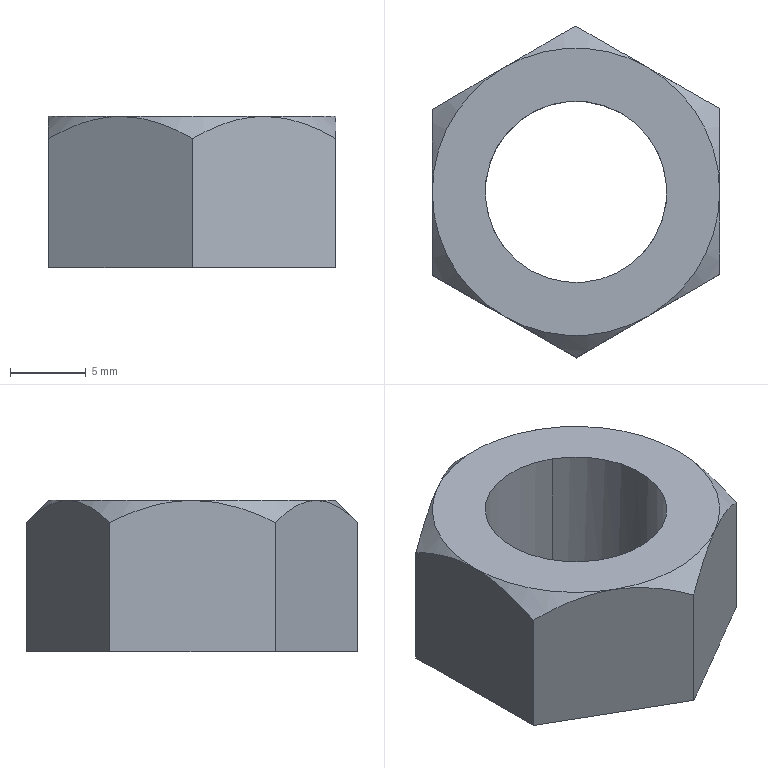Component | SolidWorks | FBR60_12_70-1_FBR12nut-1 | 1 solid | 16 faces | box 19.04 x 21.94 x 10 mm | volume 1982 mm3 | plane 8 | cone 6 | cylinder 2 | commonest cylinder face diameters 12 x2
STEP:
#1=CARTESIAN_POINT('',(-2.696,-29.611,-18.54));
#2=VERTEX_POINT('',#1);
#3=CARTESIAN_POINT('',(-2.462,-29.201,-18.54));
#4=VERTEX_POINT('',#3);
#5=CARTESIAN_POINT('',(-2.696,-29.611,-18.54));
#6=CARTESIAN_POINT('',(-2.669,-29.626,-18.54));
#7=CARTESIAN_POINT('',(-2.64,-29.636,-18.54));
#8=CARTESIAN_POINT('',(-2.578,-29.644,-18.54));
#9=CARTESIAN_POINT('',(-2.547,-29.642,-18.54));
#10=CARTESIAN_POINT('',(-2.487,-29.626,-18.54));
#11=CARTESIAN_POINT('',(-2.459,-29.612,-18.54));
#12=CARTESIAN_POINT('',(-2.41,-29.574,-18.54));
#13=CARTESIAN_POINT('',(-2.389,-29.55,-18.54));
#14=CARTESIAN_POINT('',(-2.359,-29.497,-18.54));
#15=CARTESIAN_POINT('',(-2.349,-29.467,-18.54));
#16=CARTESIAN_POINT('',(-2.341,-29.405,-18.54));
#17=CARTESIAN_POINT('',(-2.343,-29.374,-18.54));
#18=CARTESIAN_POINT('',(-2.359,-29.314,-18.54));
#19=CARTESIAN_POINT('',(-2.373,-29.286,-18.54));
#20=CARTESIAN_POINT('',(-2.402,-29.249,-18.54));
#21=CARTESIAN_POINT('',(-2.412,-29.238,-18.54));
#22=CARTESIAN_POINT('',(-2.436,-29.218,-18.54));
#23=CARTESIAN_POINT('',(-2.448,-29.209,-18.54));
#24=CARTESIAN_POINT('',(-2.462,-29.201,-18.54));
#25=B_SPLINE_CURVE_WITH_KNOTS('',3,(#5,#6,#7,#8,#9,#10,#11,#12,#13,#14,#15,#16,#17,#18,#19,#20,#21,#22,#23,#24),.UNSPECIFIED.,.F.,.F.,(4,2,2,2,2,2,2,2,2,4),(0.5,0.5625,0.625,0.6875,0.75,0.8125,0.875,0.9375,0.9688,1.),.UNSPECIFIED.);
#26=EDGE_CURVE('',#2,#4,#25,.T.);
#27=ORIENTED_EDGE('',*,*,#26,.F.);
#28=CARTESIAN_POINT('',(-2.696,-29.611,-18.147));
#29=VERTEX_POINT('',#28);
#30=CARTESIAN_POINT('',(-2.696,-29.611,-18.54));
#31=DIRECTION('',(0.,-0.,1.));
#32=VECTOR('',#31,39.37);
#33=LINE('',#30,#32);
#34=EDGE_CURVE('',#2,#29,#33,.T.);
#35=ORIENTED_EDGE('',*,*,#34,.T.);
#36=CARTESIAN_POINT('',(-2.462,-29.201,-18.147));
#37=VERTEX_POINT('',#36);
#38=CARTESIAN_POINT('',(-2.579,-29.406,-18.147));
#39=DIRECTION('',(0.,-0.,1.));
#40=DIRECTION('',(0.4969,0.8678,0.));
#41=AXIS2_PLACEMENT_3D('',#38,#39,#40);
#42=CIRCLE('',#41,0.2362);
#43=EDGE_CURVE('',#29,#37,#42,.T.);
#44=ORIENTED_EDGE('',*,*,#43,.T.);
#45=CARTESIAN_POINT('',(-2.462,-29.201,-18.54));
#46=DIRECTION('',(0.,-0.,1.));
#47=VECTOR('',#46,39.37);
#48=LINE('',#45,#47);
#49=EDGE_CURVE('',#4,#37,#48,.T.);
#50=ORIENTED_EDGE('',*,*,#49,.F.);
#51=EDGE_LOOP('',(#27,#35,#44,#50));
#52=FACE_OUTER_BOUND('',#51,.T.);
#53=CARTESIAN_POINT('',(-2.579,-29.406,-18.54));
#54=DIRECTION('',(0.,-0.,1.));
#55=DIRECTION('',(0.4969,0.8678,0.));
#56=AXIS2_PLACEMENT_3D('',#53,#54,#55);
#57=CYLINDRICAL_SURFACE('',#56,0.2362);
#58=ADVANCED_FACE('',(#52),#57,.F.);
#59=CARTESIAN_POINT('',(-2.393,-29.081,-18.147));
#60=VERTEX_POINT('',#59);
#61=CARTESIAN_POINT('',(-2.767,-29.083,-18.147));
#62=VERTEX_POINT('',#61);
#63=CARTESIAN_POINT('',(-2.579,-29.406,-18.147));
#64=DIRECTION('',(0.,-0.,1.));
#65=DIRECTION('',(0.4969,0.8678,0.));
#66=AXIS2_PLACEMENT_3D('',#63,#64,#65);
#67=CIRCLE('',#66,0.374);
#68=EDGE_CURVE('',#60,#62,#67,.T.);
#69=ORIENTED_EDGE('',*,*,#68,.T.);
#70=CARTESIAN_POINT('',(-2.953,-29.407,-18.147));
#71=VERTEX_POINT('',#70);
#72=CARTESIAN_POINT('',(-2.579,-29.406,-18.147));
#73=DIRECTION('',(0.,-0.,1.));
#74=DIRECTION('',(0.4969,0.8678,0.));
#75=AXIS2_PLACEMENT_3D('',#72,#73,#74);
#76=CIRCLE('',#75,0.374);
#77=EDGE_CURVE('',#62,#71,#76,.T.);
#78=ORIENTED_EDGE('',*,*,#77,.T.);
#79=CARTESIAN_POINT('',(-2.765,-29.731,-18.147));
#80=VERTEX_POINT('',#79);
#81=CARTESIAN_POINT('',(-2.579,-29.406,-18.147));
#82=DIRECTION('',(0.,-0.,1.));
#83=DIRECTION('',(0.4969,0.8678,0.));
#84=AXIS2_PLACEMENT_3D('',#81,#82,#83);
#85=CIRCLE('',#84,0.374);
#86=EDGE_CURVE('',#71,#80,#85,.T.);
#87=ORIENTED_EDGE('',*,*,#86,.T.);
#88=CARTESIAN_POINT('',(-2.391,-29.729,-18.147));
#89=VERTEX_POINT('',#88);
#90=CARTESIAN_POINT('',(-2.579,-29.406,-18.147));
#91=DIRECTION('',(0.,-0.,1.));
#92=DIRECTION('',(0.4969,0.8678,0.));
#93=AXIS2_PLACEMENT_3D('',#90,#91,#92);
#94=CIRCLE('',#93,0.374);
#95=EDGE_CURVE('',#80,#89,#94,.T.);
#96=ORIENTED_EDGE('',*,*,#95,.T.);
#97=CARTESIAN_POINT('',(-2.205,-29.405,-18.147));
#98=VERTEX_POINT('',#97);
#99=CARTESIAN_POINT('',(-2.579,-29.406,-18.147));
#100=DIRECTION('',(0.,-0.,1.));
#101=DIRECTION('',(0.4969,0.8678,0.));
#102=AXIS2_PLACEMENT_3D('',#99,#100,#101);
#103=CIRCLE('',#102,0.374);
#104=EDGE_CURVE('',#89,#98,#103,.T.);
#105=ORIENTED_EDGE('',*,*,#104,.T.);
#106=CARTESIAN_POINT('',(-2.579,-29.406,-18.147));
#107=DIRECTION('',(0.,-0.,1.));
#108=DIRECTION('',(0.4969,0.8678,0.));
#109=AXIS2_PLACEMENT_3D('',#106,#107,#108);
#110=CIRCLE('',#109,0.374);
#111=EDGE_CURVE('',#98,#60,#110,.T.);
#112=ORIENTED_EDGE('',*,*,#111,.T.);
#113=EDGE_LOOP('',(#69,#78,#87,#96,#105,#112));
#114=FACE_OUTER_BOUND('',#113,.T.);
#115=CARTESIAN_POINT('',(-2.579,-29.406,-18.147));
#116=DIRECTION('',(0.,-0.,1.));
#117=DIRECTION('',(0.4969,0.8678,0.));
#118=AXIS2_PLACEMENT_3D('',#115,#116,#117);
#119=CIRCLE('',#118,0.2362);
#120=EDGE_CURVE('',#37,#29,#119,.T.);
#121=ORIENTED_EDGE('',*,*,#120,.F.);
#122=ORIENTED_EDGE('',*,*,#43,.F.);
#123=EDGE_LOOP('',(#121,#122));
#124=FACE_BOUND('',#123,.T.);
#125=CARTESIAN_POINT('',(-2.579,-29.406,-18.147));
#126=DIRECTION('',(-0.,0.,-1.));
#127=DIRECTION('',(-0.4969,-0.8678,-0.));
#128=AXIS2_PLACEMENT_3D('',#125,#126,#127);
#129=PLANE('',#128);
#130=ADVANCED_FACE('',(#114,#124),#129,.F.);
#131=CARTESIAN_POINT('',(-2.204,-29.621,-18.54));
#132=VERTEX_POINT('',#131);
#133=CARTESIAN_POINT('',(-2.206,-29.189,-18.54));
#134=VERTEX_POINT('',#133);
#135=CARTESIAN_POINT('',(-2.204,-29.621,-18.54));
#136=DIRECTION('',(-0.003538,1.,0.));
#137=VECTOR('',#136,39.37);
#138=LINE('',#135,#137);
#139=EDGE_CURVE('',#132,#134,#138,.T.);
#140=ORIENTED_EDGE('',*,*,#139,.F.);
#141=CARTESIAN_POINT('',(-2.577,-29.838,-18.54));
#142=VERTEX_POINT('',#141);
#143=CARTESIAN_POINT('',(-2.577,-29.838,-18.54));
#144=DIRECTION('',(0.8643,0.5031,0.));
#145=VECTOR('',#144,39.37);
#146=LINE('',#143,#145);
#147=EDGE_CURVE('',#142,#132,#146,.T.);
#148=ORIENTED_EDGE('',*,*,#147,.F.);
#149=CARTESIAN_POINT('',(-2.952,-29.623,-18.54));
#150=VERTEX_POINT('',#149);
#151=CARTESIAN_POINT('',(-2.952,-29.623,-18.54));
#152=DIRECTION('',(0.8678,-0.4969,-0.));
#153=VECTOR('',#152,39.37);
#154=LINE('',#151,#153);
#155=EDGE_CURVE('',#150,#142,#154,.T.);
#156=ORIENTED_EDGE('',*,*,#155,.F.);
#157=CARTESIAN_POINT('',(-2.954,-29.191,-18.54));
#158=VERTEX_POINT('',#157);
#159=CARTESIAN_POINT('',(-2.954,-29.191,-18.54));
#160=DIRECTION('',(0.003538,-1.,-0.));
#161=VECTOR('',#160,39.37);
#162=LINE('',#159,#161);
#163=EDGE_CURVE('',#158,#150,#162,.T.);
#164=ORIENTED_EDGE('',*,*,#163,.F.);
#165=CARTESIAN_POINT('',(-2.58,-28.974,-18.54));
#166=VERTEX_POINT('',#165);
#167=CARTESIAN_POINT('',(-2.58,-28.974,-18.54));
#168=DIRECTION('',(-0.8643,-0.5031,-0.));
#169=VECTOR('',#168,39.37);
#170=LINE('',#167,#169);
#171=EDGE_CURVE('',#166,#158,#170,.T.);
#172=ORIENTED_EDGE('',*,*,#171,.F.);
#173=CARTESIAN_POINT('',(-2.206,-29.189,-18.54));
#174=DIRECTION('',(-0.8678,0.4969,0.));
#175=VECTOR('',#174,39.37);
#176=LINE('',#173,#175);
#177=EDGE_CURVE('',#134,#166,#176,.T.);
#178=ORIENTED_EDGE('',*,*,#177,.F.);
#179=EDGE_LOOP('',(#140,#148,#156,#164,#172,#178));
#180=FACE_OUTER_BOUND('',#179,.T.);
#181=CARTESIAN_POINT('',(-2.462,-29.201,-18.54));
#182=CARTESIAN_POINT('',(-2.488,-29.186,-18.54));
#183=CARTESIAN_POINT('',(-2.518,-29.176,-18.54));
#184=CARTESIAN_POINT('',(-2.58,-29.168,-18.54));
#185=CARTESIAN_POINT('',(-2.611,-29.17,-18.54));
#186=CARTESIAN_POINT('',(-2.671,-29.186,-18.54));
#187=CARTESIAN_POINT('',(-2.699,-29.2,-18.54));
#188=CARTESIAN_POINT('',(-2.748,-29.238,-18.54));
#189=CARTESIAN_POINT('',(-2.769,-29.262,-18.54));
#190=CARTESIAN_POINT('',(-2.799,-29.316,-18.54));
#191=CARTESIAN_POINT('',(-2.809,-29.345,-18.54));
#192=CARTESIAN_POINT('',(-2.817,-29.407,-18.54));
#193=CARTESIAN_POINT('',(-2.815,-29.438,-18.54));
#194=CARTESIAN_POINT('',(-2.799,-29.498,-18.54));
#195=CARTESIAN_POINT('',(-2.785,-29.526,-18.54));
#196=CARTESIAN_POINT('',(-2.747,-29.575,-18.54));
#197=CARTESIAN_POINT('',(-2.723,-29.596,-18.54));
#198=CARTESIAN_POINT('',(-2.696,-29.611,-18.54));
#199=B_SPLINE_CURVE_WITH_KNOTS('',3,(#181,#182,#183,#184,#185,#186,#187,#188,#189,#190,#191,#192,#193,#194,#195,#196,#197,#198),.UNSPECIFIED.,.F.,.F.,(4,2,2,2,2,2,2,2,4),(0.,0.0625,0.125,0.1875,0.25,0.3125,0.375,0.4375,0.5),.UNSPECIFIED.);
#200=EDGE_CURVE('',#4,#2,#199,.T.);
#201=ORIENTED_EDGE('',*,*,#200,.T.);
#202=ORIENTED_EDGE('',*,*,#26,.T.);
#203=EDGE_LOOP('',(#201,#202));
#204=FACE_BOUND('',#203,.T.);
#205=CARTESIAN_POINT('',(-2.968,-29.183,-18.54));
#206=DIRECTION('',(0.,-0.,1.));
#207=DIRECTION('',(0.4969,0.8678,0.));
#208=AXIS2_PLACEMENT_3D('',#205,#206,#207);
#209=PLANE('',#208);
#210=ADVANCED_FACE('',(#180,#204),#209,.F.);
#211=CARTESIAN_POINT('',(-2.577,-29.838,-18.205));
#212=VERTEX_POINT('',#211);
#213=CARTESIAN_POINT('',(-2.765,-29.731,-18.147));
#214=CARTESIAN_POINT('',(-2.757,-29.735,-18.147));
#215=CARTESIAN_POINT('',(-2.748,-29.74,-18.147));
#216=CARTESIAN_POINT('',(-2.732,-29.749,-18.149));
#217=CARTESIAN_POINT('',(-2.724,-29.754,-18.15));
#218=CARTESIAN_POINT('',(-2.7,-29.768,-18.154));
#219=CARTESIAN_POINT('',(-2.684,-29.777,-18.158));
#220=CARTESIAN_POINT('',(-2.653,-29.795,-18.168));
#221=CARTESIAN_POINT('',(-2.637,-29.804,-18.174));
#222=CARTESIAN_POINT('',(-2.607,-29.821,-18.188));
#223=CARTESIAN_POINT('',(-2.592,-29.83,-18.196));
#224=CARTESIAN_POINT('',(-2.577,-29.838,-18.205));
#225=B_SPLINE_CURVE_WITH_KNOTS('',3,(#213,#214,#215,#216,#217,#218,#219,#220,#221,#222,#223,#224),.UNSPECIFIED.,.F.,.F.,(4,2,2,2,2,4),(0.01149,0.0122,0.01291,0.01433,0.01575,0.01717),.UNSPECIFIED.);
#226=EDGE_CURVE('',#80,#212,#225,.T.);
#227=ORIENTED_EDGE('',*,*,#226,.T.);
#228=CARTESIAN_POINT('',(-2.577,-29.838,-18.205));
#229=CARTESIAN_POINT('',(-2.548,-29.821,-18.188));
#230=CARTESIAN_POINT('',(-2.518,-29.803,-18.173));
#231=CARTESIAN_POINT('',(-2.472,-29.776,-18.158));
#232=CARTESIAN_POINT('',(-2.456,-29.767,-18.154));
#233=CARTESIAN_POINT('',(-2.424,-29.748,-18.148));
#234=CARTESIAN_POINT('',(-2.407,-29.739,-18.147));
#235=CARTESIAN_POINT('',(-2.391,-29.729,-18.147));
#236=B_SPLINE_CURVE_WITH_KNOTS('',3,(#228,#229,#230,#231,#232,#233,#234,#235),.UNSPECIFIED.,.F.,.F.,(4,2,2,4),(0.00000025,0.002843,0.004264,0.005686),.UNSPECIFIED.);
#237=EDGE_CURVE('',#212,#89,#236,.T.);
#238=ORIENTED_EDGE('',*,*,#237,.T.);
#239=ORIENTED_EDGE('',*,*,#95,.F.);
#240=EDGE_LOOP('',(#227,#238,#239));
#241=FACE_OUTER_BOUND('',#240,.T.);
#242=CARTESIAN_POINT('',(-2.579,-29.406,-18.222));
#243=DIRECTION('',(-0.,0.,-1.));
#244=DIRECTION('',(-0.4969,-0.8678,0.));
#245=AXIS2_PLACEMENT_3D('',#242,#243,#244);
#246=CONICAL_SURFACE('',#245,0.4488,0.7854);
#247=ADVANCED_FACE('',(#241),#246,.T.);
#248=ORIENTED_EDGE('',*,*,#104,.F.);
#249=CARTESIAN_POINT('',(-2.204,-29.621,-18.205));
#250=VERTEX_POINT('',#249);
#251=CARTESIAN_POINT('',(-2.391,-29.729,-18.147));
#252=CARTESIAN_POINT('',(-2.358,-29.71,-18.147));
#253=CARTESIAN_POINT('',(-2.326,-29.692,-18.153));
#254=CARTESIAN_POINT('',(-2.264,-29.655,-18.173));
#255=CARTESIAN_POINT('',(-2.233,-29.638,-18.188));
#256=CARTESIAN_POINT('',(-2.204,-29.621,-18.205));
#257=B_SPLINE_CURVE_WITH_KNOTS('',3,(#251,#252,#253,#254,#255,#256),.UNSPECIFIED.,.F.,.F.,(4,2,4),(0.005686,0.008509,0.01133),.UNSPECIFIED.);
#258=EDGE_CURVE('',#89,#250,#257,.T.);
#259=ORIENTED_EDGE('',*,*,#258,.T.);
#260=CARTESIAN_POINT('',(-2.204,-29.621,-18.205));
#261=CARTESIAN_POINT('',(-2.204,-29.587,-18.188));
#262=CARTESIAN_POINT('',(-2.204,-29.552,-18.173));
#263=CARTESIAN_POINT('',(-2.205,-29.498,-18.158));
#264=CARTESIAN_POINT('',(-2.205,-29.48,-18.154));
#265=CARTESIAN_POINT('',(-2.205,-29.443,-18.148));
#266=CARTESIAN_POINT('',(-2.205,-29.424,-18.147));
#267=CARTESIAN_POINT('',(-2.205,-29.405,-18.147));
#268=B_SPLINE_CURVE_WITH_KNOTS('',3,(#260,#261,#262,#263,#264,#265,#266,#267),.UNSPECIFIED.,.F.,.F.,(4,2,2,4),(0.00000025,0.002843,0.004264,0.005686),.UNSPECIFIED.);
#269=EDGE_CURVE('',#250,#98,#268,.T.);
#270=ORIENTED_EDGE('',*,*,#269,.T.);
#271=EDGE_LOOP('',(#248,#259,#270));
#272=FACE_OUTER_BOUND('',#271,.T.);
#273=CARTESIAN_POINT('',(-2.579,-29.406,-18.222));
#274=DIRECTION('',(-0.,0.,-1.));
#275=DIRECTION('',(-0.4969,-0.8678,0.));
#276=AXIS2_PLACEMENT_3D('',#273,#274,#275);
#277=CONICAL_SURFACE('',#276,0.4488,0.7854);
#278=ADVANCED_FACE('',(#272),#277,.T.);
#279=ORIENTED_EDGE('',*,*,#111,.F.);
#280=CARTESIAN_POINT('',(-2.206,-29.189,-18.205));
#281=VERTEX_POINT('',#280);
#282=CARTESIAN_POINT('',(-2.205,-29.405,-18.147));
#283=CARTESIAN_POINT('',(-2.205,-29.367,-18.147));
#284=CARTESIAN_POINT('',(-2.205,-29.33,-18.153));
#285=CARTESIAN_POINT('',(-2.205,-29.257,-18.173));
#286=CARTESIAN_POINT('',(-2.206,-29.223,-18.188));
#287=CARTESIAN_POINT('',(-2.206,-29.189,-18.205));
#288=B_SPLINE_CURVE_WITH_KNOTS('',3,(#282,#283,#284,#285,#286,#287),.UNSPECIFIED.,.F.,.F.,(4,2,4),(0.005686,0.008509,0.01133),.UNSPECIFIED.);
#289=EDGE_CURVE('',#98,#281,#288,.T.);
#290=ORIENTED_EDGE('',*,*,#289,.T.);
#291=CARTESIAN_POINT('',(-2.206,-29.189,-18.205));
#292=CARTESIAN_POINT('',(-2.22,-29.18,-18.196));
#293=CARTESIAN_POINT('',(-2.235,-29.172,-18.188));
#294=CARTESIAN_POINT('',(-2.266,-29.155,-18.174));
#295=CARTESIAN_POINT('',(-2.281,-29.146,-18.168));
#296=CARTESIAN_POINT('',(-2.312,-29.128,-18.158));
#297=CARTESIAN_POINT('',(-2.328,-29.119,-18.154));
#298=CARTESIAN_POINT('',(-2.352,-29.105,-18.15));
#299=CARTESIAN_POINT('',(-2.36,-29.1,-18.149));
#300=CARTESIAN_POINT('',(-2.377,-29.091,-18.147));
#301=CARTESIAN_POINT('',(-2.385,-29.086,-18.147));
#302=CARTESIAN_POINT('',(-2.393,-29.081,-18.147));
#303=B_SPLINE_CURVE_WITH_KNOTS('',3,(#291,#292,#293,#294,#295,#296,#297,#298,#299,#300,#301,#302),.UNSPECIFIED.,.F.,.F.,(4,2,2,2,2,4),(0.007344,0.008765,0.01019,0.01161,0.01232,0.01303),.UNSPECIFIED.);
#304=EDGE_CURVE('',#281,#60,#303,.T.);
#305=ORIENTED_EDGE('',*,*,#304,.T.);
#306=EDGE_LOOP('',(#279,#290,#305));
#307=FACE_OUTER_BOUND('',#306,.T.);
#308=CARTESIAN_POINT('',(-2.579,-29.406,-18.222));
#309=DIRECTION('',(-0.,0.,-1.));
#310=DIRECTION('',(-0.4969,-0.8678,0.));
#311=AXIS2_PLACEMENT_3D('',#308,#309,#310);
#312=CONICAL_SURFACE('',#311,0.4488,0.7854);
#313=ADVANCED_FACE('',(#307),#312,.T.);
#314=ORIENTED_EDGE('',*,*,#68,.F.);
#315=CARTESIAN_POINT('',(-2.58,-28.974,-18.205));
#316=VERTEX_POINT('',#315);
#317=CARTESIAN_POINT('',(-2.393,-29.081,-18.147));
#318=CARTESIAN_POINT('',(-2.426,-29.063,-18.147));
#319=CARTESIAN_POINT('',(-2.458,-29.044,-18.153));
#320=CARTESIAN_POINT('',(-2.505,-29.017,-18.168));
#321=CARTESIAN_POINT('',(-2.521,-29.008,-18.174));
#322=CARTESIAN_POINT('',(-2.551,-28.991,-18.188));
#323=CARTESIAN_POINT('',(-2.566,-28.982,-18.196));
#324=CARTESIAN_POINT('',(-2.58,-28.974,-18.205));
#325=B_SPLINE_CURVE_WITH_KNOTS('',3,(#317,#318,#319,#320,#321,#322,#323,#324),.UNSPECIFIED.,.F.,.F.,(4,2,2,4),(0.01303,0.01587,0.0173,0.01872),.UNSPECIFIED.);
#326=EDGE_CURVE('',#60,#316,#325,.T.);
#327=ORIENTED_EDGE('',*,*,#326,.T.);
#328=CARTESIAN_POINT('',(-2.58,-28.974,-18.205));
#329=CARTESIAN_POINT('',(-2.61,-28.991,-18.188));
#330=CARTESIAN_POINT('',(-2.64,-29.009,-18.173));
#331=CARTESIAN_POINT('',(-2.686,-29.036,-18.158));
#332=CARTESIAN_POINT('',(-2.702,-29.045,-18.154));
#333=CARTESIAN_POINT('',(-2.734,-29.064,-18.148));
#334=CARTESIAN_POINT('',(-2.751,-29.073,-18.147));
#335=CARTESIAN_POINT('',(-2.767,-29.083,-18.147));
#336=B_SPLINE_CURVE_WITH_KNOTS('',3,(#328,#329,#330,#331,#332,#333,#334,#335),.UNSPECIFIED.,.F.,.F.,(4,2,2,4),(0.00000025,0.002843,0.004264,0.005686),.UNSPECIFIED.);
#337=EDGE_CURVE('',#316,#62,#336,.T.);
#338=ORIENTED_EDGE('',*,*,#337,.T.);
#339=EDGE_LOOP('',(#314,#327,#338));
#340=FACE_OUTER_BOUND('',#339,.T.);
#341=CARTESIAN_POINT('',(-2.579,-29.406,-18.222));
#342=DIRECTION('',(-0.,0.,-1.));
#343=DIRECTION('',(-0.4969,-0.8678,0.));
#344=AXIS2_PLACEMENT_3D('',#341,#342,#343);
#345=CONICAL_SURFACE('',#344,0.4488,0.7854);
#346=ADVANCED_FACE('',(#340),#345,.T.);
#347=ORIENTED_EDGE('',*,*,#77,.F.);
#348=CARTESIAN_POINT('',(-2.954,-29.191,-18.205));
#349=VERTEX_POINT('',#348);
#350=CARTESIAN_POINT('',(-2.767,-29.083,-18.147));
#351=CARTESIAN_POINT('',(-2.8,-29.102,-18.147));
#352=CARTESIAN_POINT('',(-2.831,-29.12,-18.153));
#353=CARTESIAN_POINT('',(-2.894,-29.157,-18.173));
#354=CARTESIAN_POINT('',(-2.925,-29.174,-18.188));
#355=CARTESIAN_POINT('',(-2.954,-29.191,-18.205));
#356=B_SPLINE_CURVE_WITH_KNOTS('',3,(#350,#351,#352,#353,#354,#355),.UNSPECIFIED.,.F.,.F.,(4,2,4),(0.005686,0.008509,0.01133),.UNSPECIFIED.);
#357=EDGE_CURVE('',#62,#349,#356,.T.);
#358=ORIENTED_EDGE('',*,*,#357,.T.);
#359=CARTESIAN_POINT('',(-2.954,-29.191,-18.205));
#360=CARTESIAN_POINT('',(-2.954,-29.225,-18.188));
#361=CARTESIAN_POINT('',(-2.953,-29.26,-18.173));
#362=CARTESIAN_POINT('',(-2.953,-29.314,-18.158));
#363=CARTESIAN_POINT('',(-2.953,-29.332,-18.154));
#364=CARTESIAN_POINT('',(-2.953,-29.369,-18.148));
#365=CARTESIAN_POINT('',(-2.953,-29.388,-18.147));
#366=CARTESIAN_POINT('',(-2.953,-29.407,-18.147));
#367=B_SPLINE_CURVE_WITH_KNOTS('',3,(#359,#360,#361,#362,#363,#364,#365,#366),.UNSPECIFIED.,.F.,.F.,(4,2,2,4),(0.00000025,0.002843,0.004264,0.005686),.UNSPECIFIED.);
#368=EDGE_CURVE('',#349,#71,#367,.T.);
#369=ORIENTED_EDGE('',*,*,#368,.T.);
#370=EDGE_LOOP('',(#347,#358,#369));
#371=FACE_OUTER_BOUND('',#370,.T.);
#372=CARTESIAN_POINT('',(-2.579,-29.406,-18.222));
#373=DIRECTION('',(-0.,0.,-1.));
#374=DIRECTION('',(-0.4969,-0.8678,0.));
#375=AXIS2_PLACEMENT_3D('',#372,#373,#374);
#376=CONICAL_SURFACE('',#375,0.4488,0.7854);
#377=ADVANCED_FACE('',(#371),#376,.T.);
#378=ORIENTED_EDGE('',*,*,#86,.F.);
#379=CARTESIAN_POINT('',(-2.952,-29.623,-18.205));
#380=VERTEX_POINT('',#379);
#381=CARTESIAN_POINT('',(-2.953,-29.407,-18.147));
#382=CARTESIAN_POINT('',(-2.953,-29.445,-18.147));
#383=CARTESIAN_POINT('',(-2.953,-29.482,-18.153));
#384=CARTESIAN_POINT('',(-2.952,-29.555,-18.173));
#385=CARTESIAN_POINT('',(-2.952,-29.589,-18.188));
#386=CARTESIAN_POINT('',(-2.952,-29.623,-18.205));
#387=B_SPLINE_CURVE_WITH_KNOTS('',3,(#381,#382,#383,#384,#385,#386),.UNSPECIFIED.,.F.,.F.,(4,2,4),(0.005686,0.008509,0.01133),.UNSPECIFIED.);
#388=EDGE_CURVE('',#71,#380,#387,.T.);
#389=ORIENTED_EDGE('',*,*,#388,.T.);
#390=CARTESIAN_POINT('',(-2.952,-29.623,-18.205));
#391=CARTESIAN_POINT('',(-2.938,-29.632,-18.196));
#392=CARTESIAN_POINT('',(-2.923,-29.64,-18.188));
#393=CARTESIAN_POINT('',(-2.893,-29.657,-18.174));
#394=CARTESIAN_POINT('',(-2.877,-29.666,-18.168));
#395=CARTESIAN_POINT('',(-2.83,-29.693,-18.153));
#396=CARTESIAN_POINT('',(-2.798,-29.712,-18.147));
#397=CARTESIAN_POINT('',(-2.765,-29.731,-18.147));
#398=B_SPLINE_CURVE_WITH_KNOTS('',3,(#390,#391,#392,#393,#394,#395,#396,#397),.UNSPECIFIED.,.F.,.F.,(4,2,2,4),(0.005801,0.007223,0.008644,0.01149),.UNSPECIFIED.);
#399=EDGE_CURVE('',#380,#80,#398,.T.);
#400=ORIENTED_EDGE('',*,*,#399,.T.);
#401=EDGE_LOOP('',(#378,#389,#400));
#402=FACE_OUTER_BOUND('',#401,.T.);
#403=CARTESIAN_POINT('',(-2.579,-29.406,-18.222));
#404=DIRECTION('',(-0.,0.,-1.));
#405=DIRECTION('',(-0.4969,-0.8678,0.));
#406=AXIS2_PLACEMENT_3D('',#403,#404,#405);
#407=CONICAL_SURFACE('',#406,0.4488,0.7854);
#408=ADVANCED_FACE('',(#402),#407,.T.);
#409=CARTESIAN_POINT('',(-2.577,-29.838,-18.107));
#410=DIRECTION('',(-0.,0.,-1.));
#411=VECTOR('',#410,39.37);
#412=LINE('',#409,#411);
#413=EDGE_CURVE('',#212,#142,#412,.T.);
#414=ORIENTED_EDGE('',*,*,#413,.T.);
#415=ORIENTED_EDGE('',*,*,#147,.T.);
#416=CARTESIAN_POINT('',(-2.204,-29.621,-18.107));
#417=DIRECTION('',(-0.,0.,-1.));
#418=VECTOR('',#417,39.37);
#419=LINE('',#416,#418);
#420=EDGE_CURVE('',#250,#132,#419,.T.);
#421=ORIENTED_EDGE('',*,*,#420,.F.);
#422=ORIENTED_EDGE('',*,*,#258,.F.);
#423=ORIENTED_EDGE('',*,*,#237,.F.);
#424=EDGE_LOOP('',(#414,#415,#421,#422,#423));
#425=FACE_OUTER_BOUND('',#424,.T.);
#426=CARTESIAN_POINT('',(-2.577,-29.838,-18.107));
#427=DIRECTION('',(-0.5031,0.8643,0.));
#428=DIRECTION('',(-0.8643,-0.5031,-0.));
#429=AXIS2_PLACEMENT_3D('',#426,#427,#428);
#430=PLANE('',#429);
#431=ADVANCED_FACE('',(#425),#430,.F.);
#432=ORIENTED_EDGE('',*,*,#420,.T.);
#433=ORIENTED_EDGE('',*,*,#139,.T.);
#434=CARTESIAN_POINT('',(-2.206,-29.189,-18.107));
#435=DIRECTION('',(-0.,0.,-1.));
#436=VECTOR('',#435,39.37);
#437=LINE('',#434,#436);
#438=EDGE_CURVE('',#281,#134,#437,.T.);
#439=ORIENTED_EDGE('',*,*,#438,.F.);
#440=ORIENTED_EDGE('',*,*,#289,.F.);
#441=ORIENTED_EDGE('',*,*,#269,.F.);
#442=EDGE_LOOP('',(#432,#433,#439,#440,#441));
#443=FACE_OUTER_BOUND('',#442,.T.);
#444=CARTESIAN_POINT('',(-2.204,-29.621,-18.107));
#445=DIRECTION('',(-1.,-0.003538,0.));
#446=DIRECTION('',(0.003538,-1.,-0.));
#447=AXIS2_PLACEMENT_3D('',#444,#445,#446);
#448=PLANE('',#447);
#449=ADVANCED_FACE('',(#443),#448,.F.);
#450=ORIENTED_EDGE('',*,*,#438,.T.);
#451=ORIENTED_EDGE('',*,*,#177,.T.);
#452=CARTESIAN_POINT('',(-2.58,-28.974,-18.107));
#453=DIRECTION('',(-0.,0.,-1.));
#454=VECTOR('',#453,39.37);
#455=LINE('',#452,#454);
#456=EDGE_CURVE('',#316,#166,#455,.T.);
#457=ORIENTED_EDGE('',*,*,#456,.F.);
#458=ORIENTED_EDGE('',*,*,#326,.F.);
#459=ORIENTED_EDGE('',*,*,#304,.F.);
#460=EDGE_LOOP('',(#450,#451,#457,#458,#459));
#461=FACE_OUTER_BOUND('',#460,.T.);
#462=CARTESIAN_POINT('',(-2.206,-29.189,-18.107));
#463=DIRECTION('',(-0.4969,-0.8678,-0.));
#464=DIRECTION('',(0.8678,-0.4969,-0.));
#465=AXIS2_PLACEMENT_3D('',#462,#463,#464);
#466=PLANE('',#465);
#467=ADVANCED_FACE('',(#461),#466,.F.);
#468=ORIENTED_EDGE('',*,*,#456,.T.);
#469=ORIENTED_EDGE('',*,*,#171,.T.);
#470=CARTESIAN_POINT('',(-2.954,-29.191,-18.107));
#471=DIRECTION('',(-0.,0.,-1.));
#472=VECTOR('',#471,39.37);
#473=LINE('',#470,#472);
#474=EDGE_CURVE('',#349,#158,#473,.T.);
#475=ORIENTED_EDGE('',*,*,#474,.F.);
#476=ORIENTED_EDGE('',*,*,#357,.F.);
#477=ORIENTED_EDGE('',*,*,#337,.F.);
#478=EDGE_LOOP('',(#468,#469,#475,#476,#477));
#479=FACE_OUTER_BOUND('',#478,.T.);
#480=CARTESIAN_POINT('',(-2.58,-28.974,-18.107));
#481=DIRECTION('',(0.5031,-0.8643,-0.));
#482=DIRECTION('',(0.8643,0.5031,0.));
#483=AXIS2_PLACEMENT_3D('',#480,#481,#482);
#484=PLANE('',#483);
#485=ADVANCED_FACE('',(#479),#484,.F.);
#486=ORIENTED_EDGE('',*,*,#474,.T.);
#487=ORIENTED_EDGE('',*,*,#163,.T.);
#488=CARTESIAN_POINT('',(-2.952,-29.623,-18.107));
#489=DIRECTION('',(-0.,0.,-1.));
#490=VECTOR('',#489,39.37);
#491=LINE('',#488,#490);
#492=EDGE_CURVE('',#380,#150,#491,.T.);
#493=ORIENTED_EDGE('',*,*,#492,.F.);
#494=ORIENTED_EDGE('',*,*,#388,.F.);
#495=ORIENTED_EDGE('',*,*,#368,.F.);
#496=EDGE_LOOP('',(#486,#487,#493,#494,#495));
#497=FACE_OUTER_BOUND('',#496,.T.);
#498=CARTESIAN_POINT('',(-2.954,-29.191,-18.107));
#499=DIRECTION('',(1.,0.003538,-0.));
#500=DIRECTION('',(-0.003538,1.,0.));
#501=AXIS2_PLACEMENT_3D('',#498,#499,#500);
#502=PLANE('',#501);
#503=ADVANCED_FACE('',(#497),#502,.F.);
#504=ORIENTED_EDGE('',*,*,#492,.T.);
#505=ORIENTED_EDGE('',*,*,#155,.T.);
#506=ORIENTED_EDGE('',*,*,#413,.F.);
#507=ORIENTED_EDGE('',*,*,#226,.F.);
#508=ORIENTED_EDGE('',*,*,#399,.F.);
#509=EDGE_LOOP('',(#504,#505,#506,#507,#508));
#510=FACE_OUTER_BOUND('',#509,.T.);
#511=CARTESIAN_POINT('',(-2.952,-29.623,-18.107));
#512=DIRECTION('',(0.4969,0.8678,0.));
#513=DIRECTION('',(-0.8678,0.4969,0.));
#514=AXIS2_PLACEMENT_3D('',#511,#512,#513);
#515=PLANE('',#514);
#516=ADVANCED_FACE('',(#510),#515,.F.);
#517=ORIENTED_EDGE('',*,*,#34,.F.);
#518=ORIENTED_EDGE('',*,*,#200,.F.);
#519=ORIENTED_EDGE('',*,*,#49,.T.);
#520=ORIENTED_EDGE('',*,*,#120,.T.);
#521=EDGE_LOOP('',(#517,#518,#519,#520));
#522=FACE_OUTER_BOUND('',#521,.T.);
#523=CARTESIAN_POINT('',(-2.579,-29.406,-18.54));
#524=DIRECTION('',(0.,-0.,1.));
#525=DIRECTION('',(0.4969,0.8678,0.));
#526=AXIS2_PLACEMENT_3D('',#523,#524,#525);
#527=CYLINDRICAL_SURFACE('',#526,0.2362);
#528=ADVANCED_FACE('',(#522),#527,.F.);
#529=CLOSED_SHELL('',(#58,#130,#210,#247,#278,#313,#346,#377,#408,#431,#449,#467,#485,#503,#516,#528));
#530=MANIFOLD_SOLID_BREP('',#529);
#531=CARTESIAN_POINT('',(0.,0.,0.));
#532=DIRECTION('',(0.,0.,1.));
#533=DIRECTION('',(1.,0.,0.));
#534=AXIS2_PLACEMENT_3D('',#531,#532,#533);
#535=(LENGTH_UNIT()NAMED_UNIT(*)SI_UNIT($,.METRE.));
#536=LENGTH_MEASURE_WITH_UNIT(LENGTH_MEASURE(0.0254),#535);
#537=DIMENSIONAL_EXPONENTS(1.,0.,0.,0.,0.,0.,0.);
#538=(CONVERSION_BASED_UNIT('',#536)LENGTH_UNIT()NAMED_UNIT(#537));
#539=UNCERTAINTY_MEASURE_WITH_UNIT(LENGTH_MEASURE(0.00001),#538,'','');
#540=(NAMED_UNIT(*)PLANE_ANGLE_UNIT()SI_UNIT($,.RADIAN.));
#541=(NAMED_UNIT(*)SI_UNIT($,.STERADIAN.)SOLID_ANGLE_UNIT());
#542=(GEOMETRIC_REPRESENTATION_CONTEXT(3)GLOBAL_UNCERTAINTY_ASSIGNED_CONTEXT((#539))GLOBAL_UNIT_ASSIGNED_CONTEXT((#538,#540,#541))REPRESENTATION_CONTEXT('',''));
#543=ADVANCED_BREP_SHAPE_REPRESENTATION('',(#530,#534),#542);
#544=COLOUR_RGB('',0.7922,0.8196,0.9333);
#545=FILL_AREA_STYLE_COLOUR('',#544);
#546=FILL_AREA_STYLE('',(#545));
#547=SURFACE_STYLE_FILL_AREA(#546);
#548=SURFACE_SIDE_STYLE('',(#547));
#549=SURFACE_STYLE_USAGE(.BOTH.,#548);
#550=PRESENTATION_STYLE_ASSIGNMENT((#549));
#551=STYLED_ITEM('',(#550),#530);
#552=PRESENTATION_LAYER_ASSIGNMENT('','',(#551));
#553=(LENGTH_UNIT()NAMED_UNIT(*)SI_UNIT($,.METRE.));
#554=LENGTH_MEASURE_WITH_UNIT(LENGTH_MEASURE(0.0254),#553);
#555=DIMENSIONAL_EXPONENTS(1.,0.,0.,0.,0.,0.,0.);
#556=(CONVERSION_BASED_UNIT('',#554)LENGTH_UNIT()NAMED_UNIT(#555));
#557=UNCERTAINTY_MEASURE_WITH_UNIT(LENGTH_MEASURE(0.00001),#556,'','');
#558=(NAMED_UNIT(*)PLANE_ANGLE_UNIT()SI_UNIT($,.RADIAN.));
#559=(NAMED_UNIT(*)SI_UNIT($,.STERADIAN.)SOLID_ANGLE_UNIT());
#560=(GEOMETRIC_REPRESENTATION_CONTEXT(3)GLOBAL_UNCERTAINTY_ASSIGNED_CONTEXT((#557))GLOBAL_UNIT_ASSIGNED_CONTEXT((#556,#558,#559))REPRESENTATION_CONTEXT('',''));
#561=MECHANICAL_DESIGN_GEOMETRIC_PRESENTATION_REPRESENTATION('',(#551),#560);